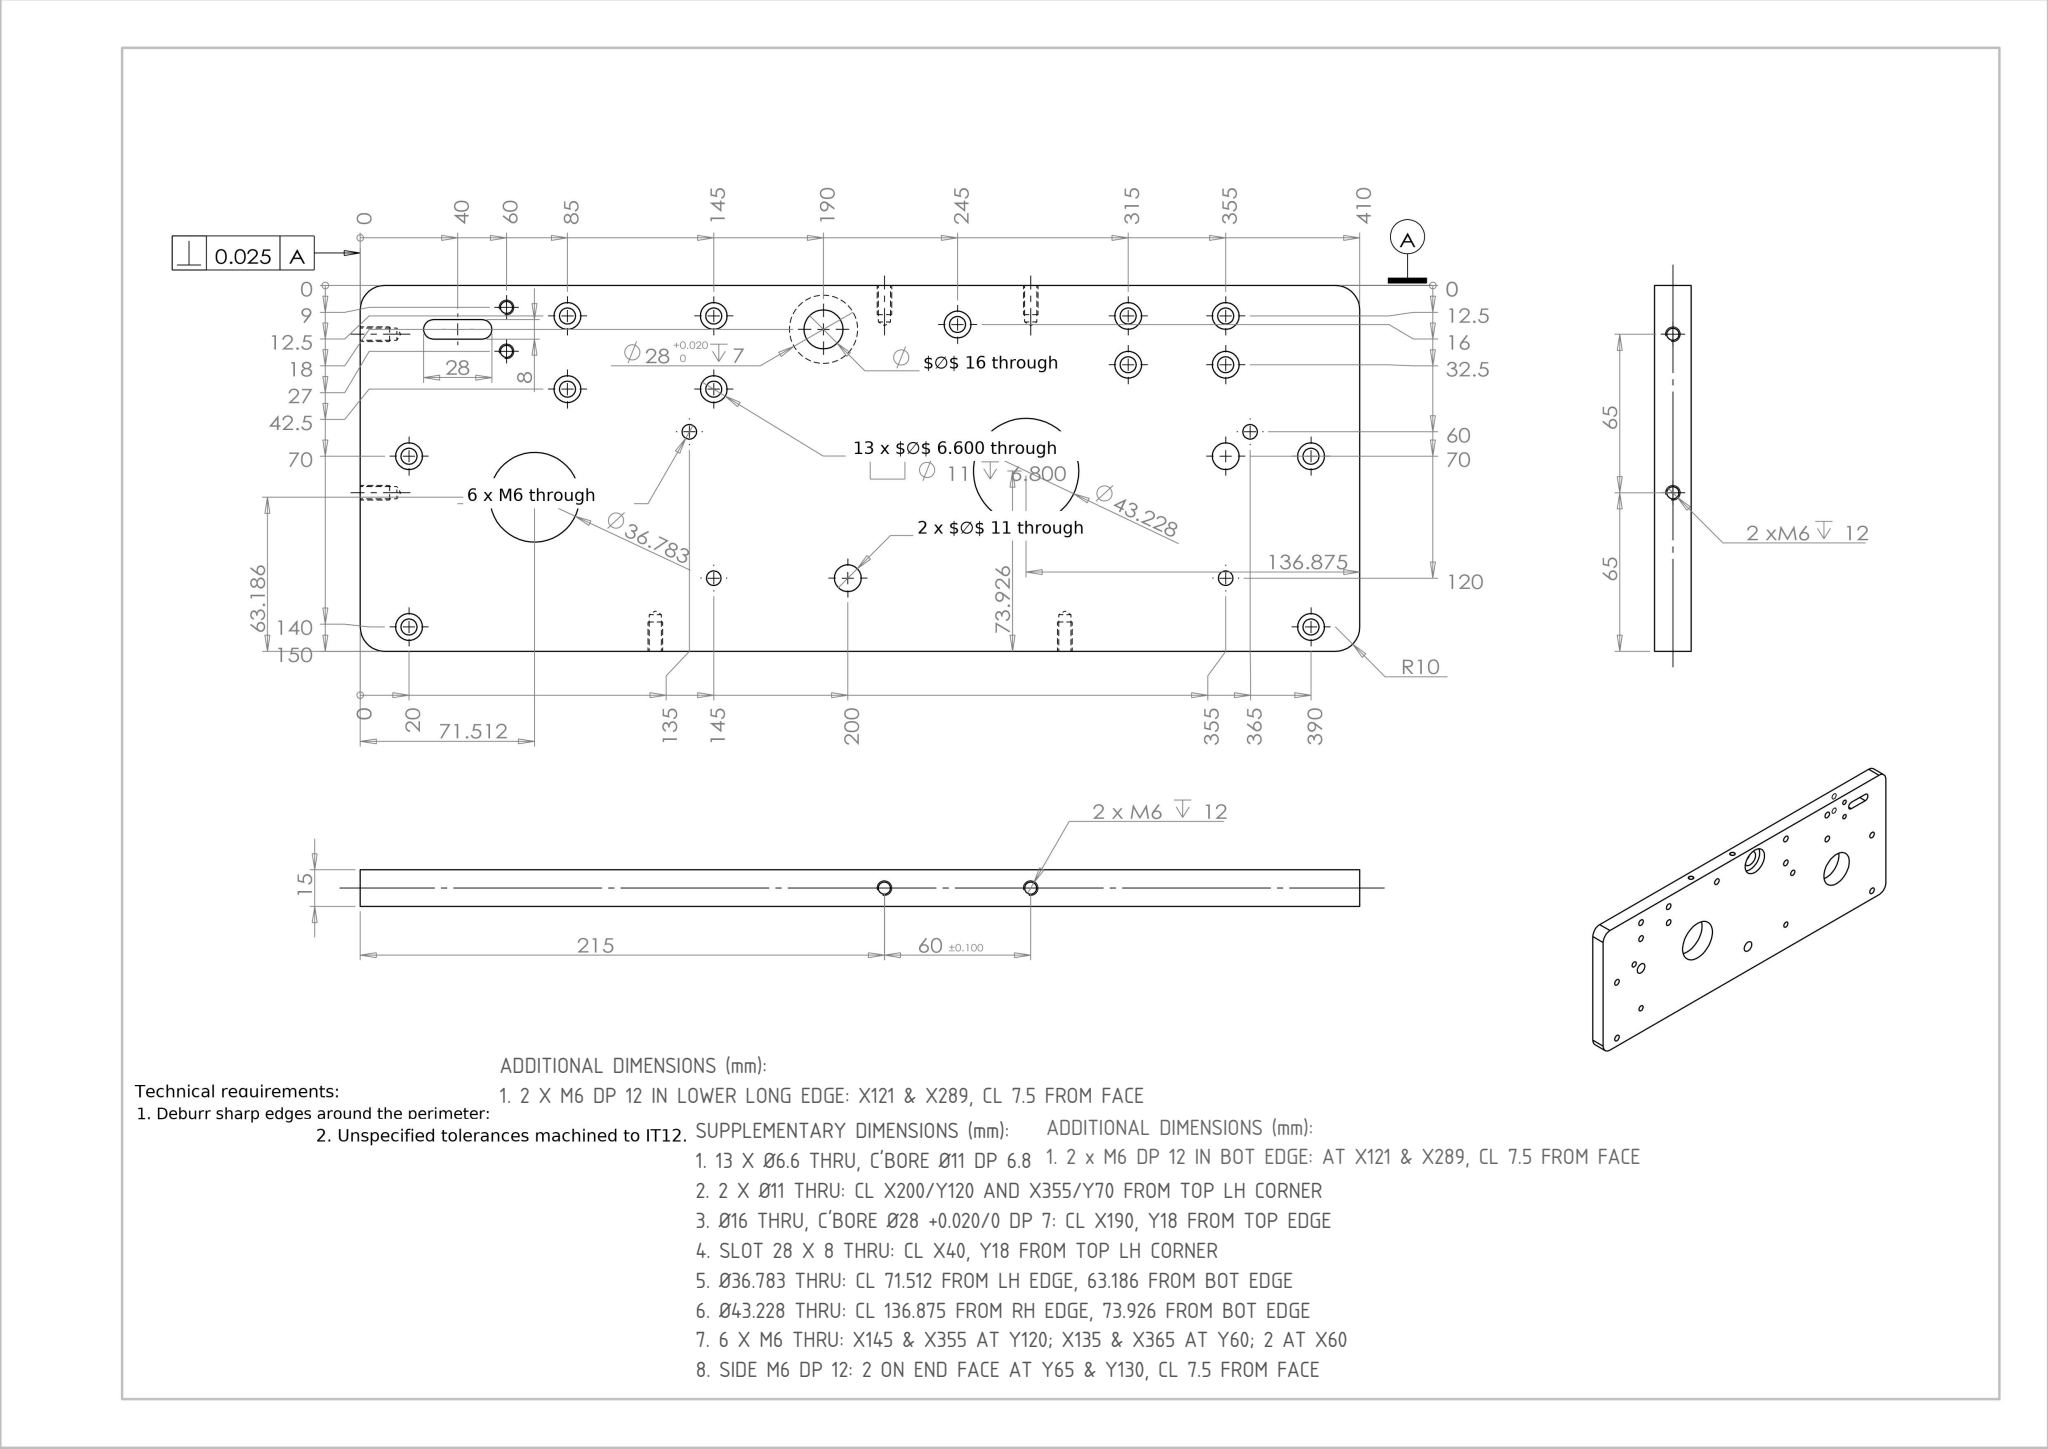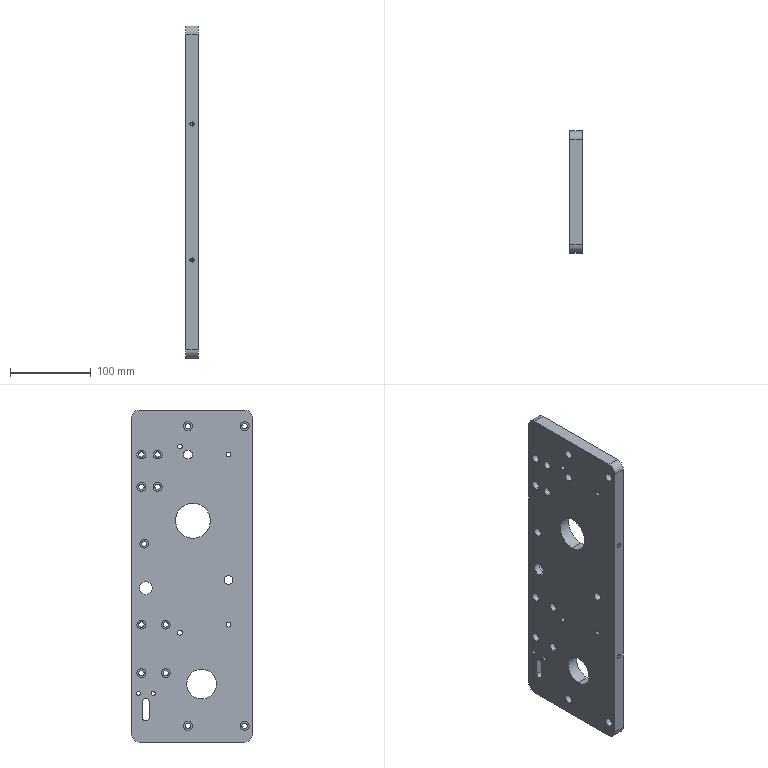Part | SolidWorks | mm | 1 solid | 129 faces | box 15 x 150 x 410 mm | volume 855175 mm3 | cylinder 95 | plane 22 | cone 12 | commonest cylinder face diameters 11 x30 6.6 x26 5 x16 6 x8 20 x4 8 x3 43.228 x2 36.783 x2
build123d program:
from build123d import *

# Parameters (mm, degrees)
BOSS_EXTRUDE1_DEPTH                                  = 15
F_16_0_16_DIAMETER_HOLE2_D                           = 16
CUT_EXTRUDE1_DEPTH                                   = 391.288
M6_TAPPED_HOLE6_D                                    = 5
HOLE_SIZE_ACCORDING_TO_THE_TYPE_6_OF_HEX_D           = 6.6
HOLE_SIZE_ACCORDING_TO_THE_TYPE_6_OF_HEX_CBORE_D     = 11
HOLE_SIZE_ACCORDING_TO_THE_TYPE_6_OF_HEX_CBORE_DEPTH = 6.8
HOLE_SIZE_ACCORDING_TO_THE_TYPE_4_OF_HEX_D           = 6.6
HOLE_SIZE_ACCORDING_TO_THE_TYPE_4_OF_HEX_CBORE_D     = 11
HOLE_SIZE_ACCORDING_TO_THE_TYPE_4_OF_HEX_CBORE_DEPTH = 6.8
SKETCH27_R                                           = 14
CUT_EXTRUDE2_DEPTH                                   = 7
SKETCH33_W                                           = 15
SKETCH33_H                                           = 150
BOSS_EXTRUDE3_DEPTH                                  = 10
M6_TAPPED_HOLE8_D                                    = 5
M6_TAPPED_HOLE8_DEPTH                                = 15
M6_TAPPED_HOLE8_TIP                                  = 1.502
SKETCH36_W                                           = 15
SKETCH36_H                                           = 150
BOSS_EXTRUDE4_DEPTH                                  = 40
HOLE_SIZE_ACCORDING_TO_THE_TYPE_5_OF_HEX_D           = 6.6
HOLE_SIZE_ACCORDING_TO_THE_TYPE_5_OF_HEX_CBORE_D     = 11
HOLE_SIZE_ACCORDING_TO_THE_TYPE_5_OF_HEX_CBORE_DEPTH = 6.8
M6_TAPPED_HOLE9_D                                    = 5
M6_TAPPED_HOLE9_DEPTH                                = 15
M6_TAPPED_HOLE9_TIP                                  = 1.502
HOLE_SIZE_ACCORDING_TO_THE_TYPE_6_OF_2_D             = 6.6
HOLE_SIZE_ACCORDING_TO_THE_TYPE_6_OF_2_CBORE_D       = 11
HOLE_SIZE_ACCORDING_TO_THE_TYPE_6_OF_2_CBORE_DEPTH   = 6.8
FILLET1_R                                            = 10
LPATTERN1_COUNT                                      = 2
LPATTERN1_PITCH                                      = 370
M6_TAPPED_HOLE10_D                                   = 6
F_11_0_11_DIAMETER_HOLE1_D                           = 11
M6_TAPPED_HOLE11_D                                   = 5
M6_TAPPED_HOLE11_DEPTH                               = 15
M6_TAPPED_HOLE11_TIP                                 = 1.502
SKETCH49_R                                           = 21.614
SKETCH49_R_2                                         = 18.392
CUT_EXTRUDE3_DEPTH                                   = 92


with BuildPart() as part:
    # Sketch1 → Boss-Extrude1 (new body)
    with BuildSketch(Plane(origin=(0, 0, 0), x_dir=(0, 0, -1), z_dir=(1, 0, 0))):
        Polygon((0, 0), (65, 0), (360, 0), (360, 150), (0, 150), align=None)
    extrude(amount=BOSS_EXTRUDE1_DEPTH)

    # 16.0 _16_ Diameter Hole2 (through all)
    with Locations(Plane(origin=(15, 0, 0), x_dir=(0, 0, -1), z_dir=(1, 0, 0))):
        with Locations((180, 132)):
            Hole(F_16_0_16_DIAMETER_HOLE2_D / 2)

    # Sketch8 → Cut-Extrude1 (cut, through all)
    with BuildSketch(Plane(origin=(15, 0, 0), x_dir=(0, 0, -1), z_dir=(1, 0, 0))):
        with BuildLine():
            Line((340, 128), (320, 128))
            ThreePointArc((320, 128), (316, 132), (320, 136))
            Line((320, 136), (340, 136))
            ThreePointArc((340, 136), (344, 132), (340, 128))
        make_face()
    extrude(amount=-CUT_EXTRUDE1_DEPTH, mode=Mode.SUBTRACT)

    # M6 Tapped Hole6 (through all)
    with Locations(Plane.ZY):
        with Locations((-310, 123), (-310, 141)):
            Hole(M6_TAPPED_HOLE6_D / 2)

    # Hole Size according to the type 6 of Hex (through all)
    with Locations(Plane.ZY):
        with Locations((-350, 80), (-350, 10)):
            hole_size_according_to_the_type_6_of_hex = CounterBoreHole(HOLE_SIZE_ACCORDING_TO_THE_TYPE_6_OF_HEX_D / 2, HOLE_SIZE_ACCORDING_TO_THE_TYPE_6_OF_HEX_CBORE_D / 2, HOLE_SIZE_ACCORDING_TO_THE_TYPE_6_OF_HEX_CBORE_DEPTH)

    # Hole Size according to the type 4 of Hex (through all)
    with Locations(Plane.ZY):
        with Locations((-285, 137.5), (-225, 137.5), (-285, 107.5), (-225, 107.5)):
            CounterBoreHole(HOLE_SIZE_ACCORDING_TO_THE_TYPE_4_OF_HEX_D / 2, HOLE_SIZE_ACCORDING_TO_THE_TYPE_4_OF_HEX_CBORE_D / 2, HOLE_SIZE_ACCORDING_TO_THE_TYPE_4_OF_HEX_CBORE_DEPTH)

    # Sketch27 → Cut-Extrude2 (cut)
    with BuildSketch(Plane(origin=(15, 0, 0), x_dir=(0, 0, -1), z_dir=(1, 0, 0))):
        with Locations((180, 132)):
            Circle(SKETCH27_R)
    extrude(amount=-CUT_EXTRUDE2_DEPTH, mode=Mode.SUBTRACT)

    # Sketch33 → Boss-Extrude3 (add)
    with BuildSketch(Plane(origin=(0, 0, -360), x_dir=(-1, 0, 0), z_dir=(0, 0, -1))):
        with Locations((-7.5, 75)):
            Rectangle(SKETCH33_W, SKETCH33_H)
    extrude(amount=BOSS_EXTRUDE3_DEPTH)

    # M6 Tapped Hole8
    with Locations(Plane(origin=(0, 0, -370), x_dir=(-1, 0, 0), z_dir=(0, 0, -1))):
        with Locations((-7.5, 130), (-7.5, 65)):
            Hole(M6_TAPPED_HOLE8_D / 2, depth=M6_TAPPED_HOLE8_DEPTH)
            with Locations((0, 0, -(M6_TAPPED_HOLE8_DEPTH + M6_TAPPED_HOLE8_TIP / 2))):  # 118° drill point
                Cone(0, M6_TAPPED_HOLE8_D / 2, M6_TAPPED_HOLE8_TIP, mode=Mode.SUBTRACT)

    # Sketch36 → Boss-Extrude4 (add)
    with BuildSketch(Plane.XY):
        with Locations((7.5, 75)):
            Rectangle(SKETCH36_W, SKETCH36_H)
    extrude(amount=BOSS_EXTRUDE4_DEPTH)

    # Hole Size according to the type 5 of Hex (through all)
    with Locations(Plane.ZY):
        with Locations((-15, 137.5), (-55, 137.5), (-15, 117.5), (-55, 117.5)):
            CounterBoreHole(HOLE_SIZE_ACCORDING_TO_THE_TYPE_5_OF_HEX_D / 2, HOLE_SIZE_ACCORDING_TO_THE_TYPE_5_OF_HEX_CBORE_D / 2, HOLE_SIZE_ACCORDING_TO_THE_TYPE_5_OF_HEX_CBORE_DEPTH)

    # M6 Tapped Hole9
    with Locations(Plane(origin=(0, 150, 0), x_dir=(-1, 0, 0), z_dir=(0, 1, 0))):
        with Locations((-7.5, -155), (-7.5, -95)):
            Hole(M6_TAPPED_HOLE9_D / 2, depth=M6_TAPPED_HOLE9_DEPTH)
            with Locations((0, 0, -(M6_TAPPED_HOLE9_DEPTH + M6_TAPPED_HOLE9_TIP / 2))):  # 118° drill point
                Cone(0, M6_TAPPED_HOLE9_D / 2, M6_TAPPED_HOLE9_TIP, mode=Mode.SUBTRACT)

    # Hole Size according to the type 6 of 2 (through all)
    with Locations(Plane.ZY):
        with Locations((-125, 134)):
            CounterBoreHole(HOLE_SIZE_ACCORDING_TO_THE_TYPE_6_OF_2_D / 2, HOLE_SIZE_ACCORDING_TO_THE_TYPE_6_OF_2_CBORE_D / 2, HOLE_SIZE_ACCORDING_TO_THE_TYPE_6_OF_2_CBORE_DEPTH)

    # Fillet1
    fillet1_edges = [part.edges().sort_by_distance(p)[0] for p in [
        (7.5, 0, 40),
        (7.5, 150, 40),
        (7.5, 0, -370),
        (7.5, 150, -370),
    ]]
    fillet(fillet1_edges, radius=FILLET1_R)

    # LPattern1: Hole Size according to the type 6 of Hex ×2
    with Locations(*[(0, 0, i * LPATTERN1_PITCH) for i in range(1, LPATTERN1_COUNT)]):
        add(hole_size_according_to_the_type_6_of_hex, mode=Mode.SUBTRACT)

    # M6 Tapped Hole10 (through all)
    with Locations(Plane.ZY):
        with Locations((-225, 30), (-5, 90), (-15, 30), (-235, 90)):
            Hole(M6_TAPPED_HOLE10_D / 2)

    # 11.0 _11_ Diameter Hole1 (through all)
    with Locations(Plane.ZY):
        with Locations((-15, 80), (-170, 30)):
            Hole(F_11_0_11_DIAMETER_HOLE1_D / 2)

    # M6 Tapped Hole11
    with Locations(Plane.XZ):
        with Locations((7.5, -249), (7.5, -81)):
            Hole(M6_TAPPED_HOLE11_D / 2, depth=M6_TAPPED_HOLE11_DEPTH)
            with Locations((0, 0, -(M6_TAPPED_HOLE11_DEPTH + M6_TAPPED_HOLE11_TIP / 2))):  # 118° drill point
                Cone(0, M6_TAPPED_HOLE11_D / 2, M6_TAPPED_HOLE11_TIP, mode=Mode.SUBTRACT)

    # Sketch49 → Cut-Extrude3 (cut)
    with BuildSketch(Plane(origin=(15, 0, 0), x_dir=(0, 0, -1), z_dir=(1, 0, 0))):
        with Locations((96.875, 73.926)):
            Circle(SKETCH49_R)
        with Locations((298.488, 63.186)):
            Circle(SKETCH49_R_2)
    extrude(amount=-CUT_EXTRUDE3_DEPTH, mode=Mode.SUBTRACT)


solid = part.part